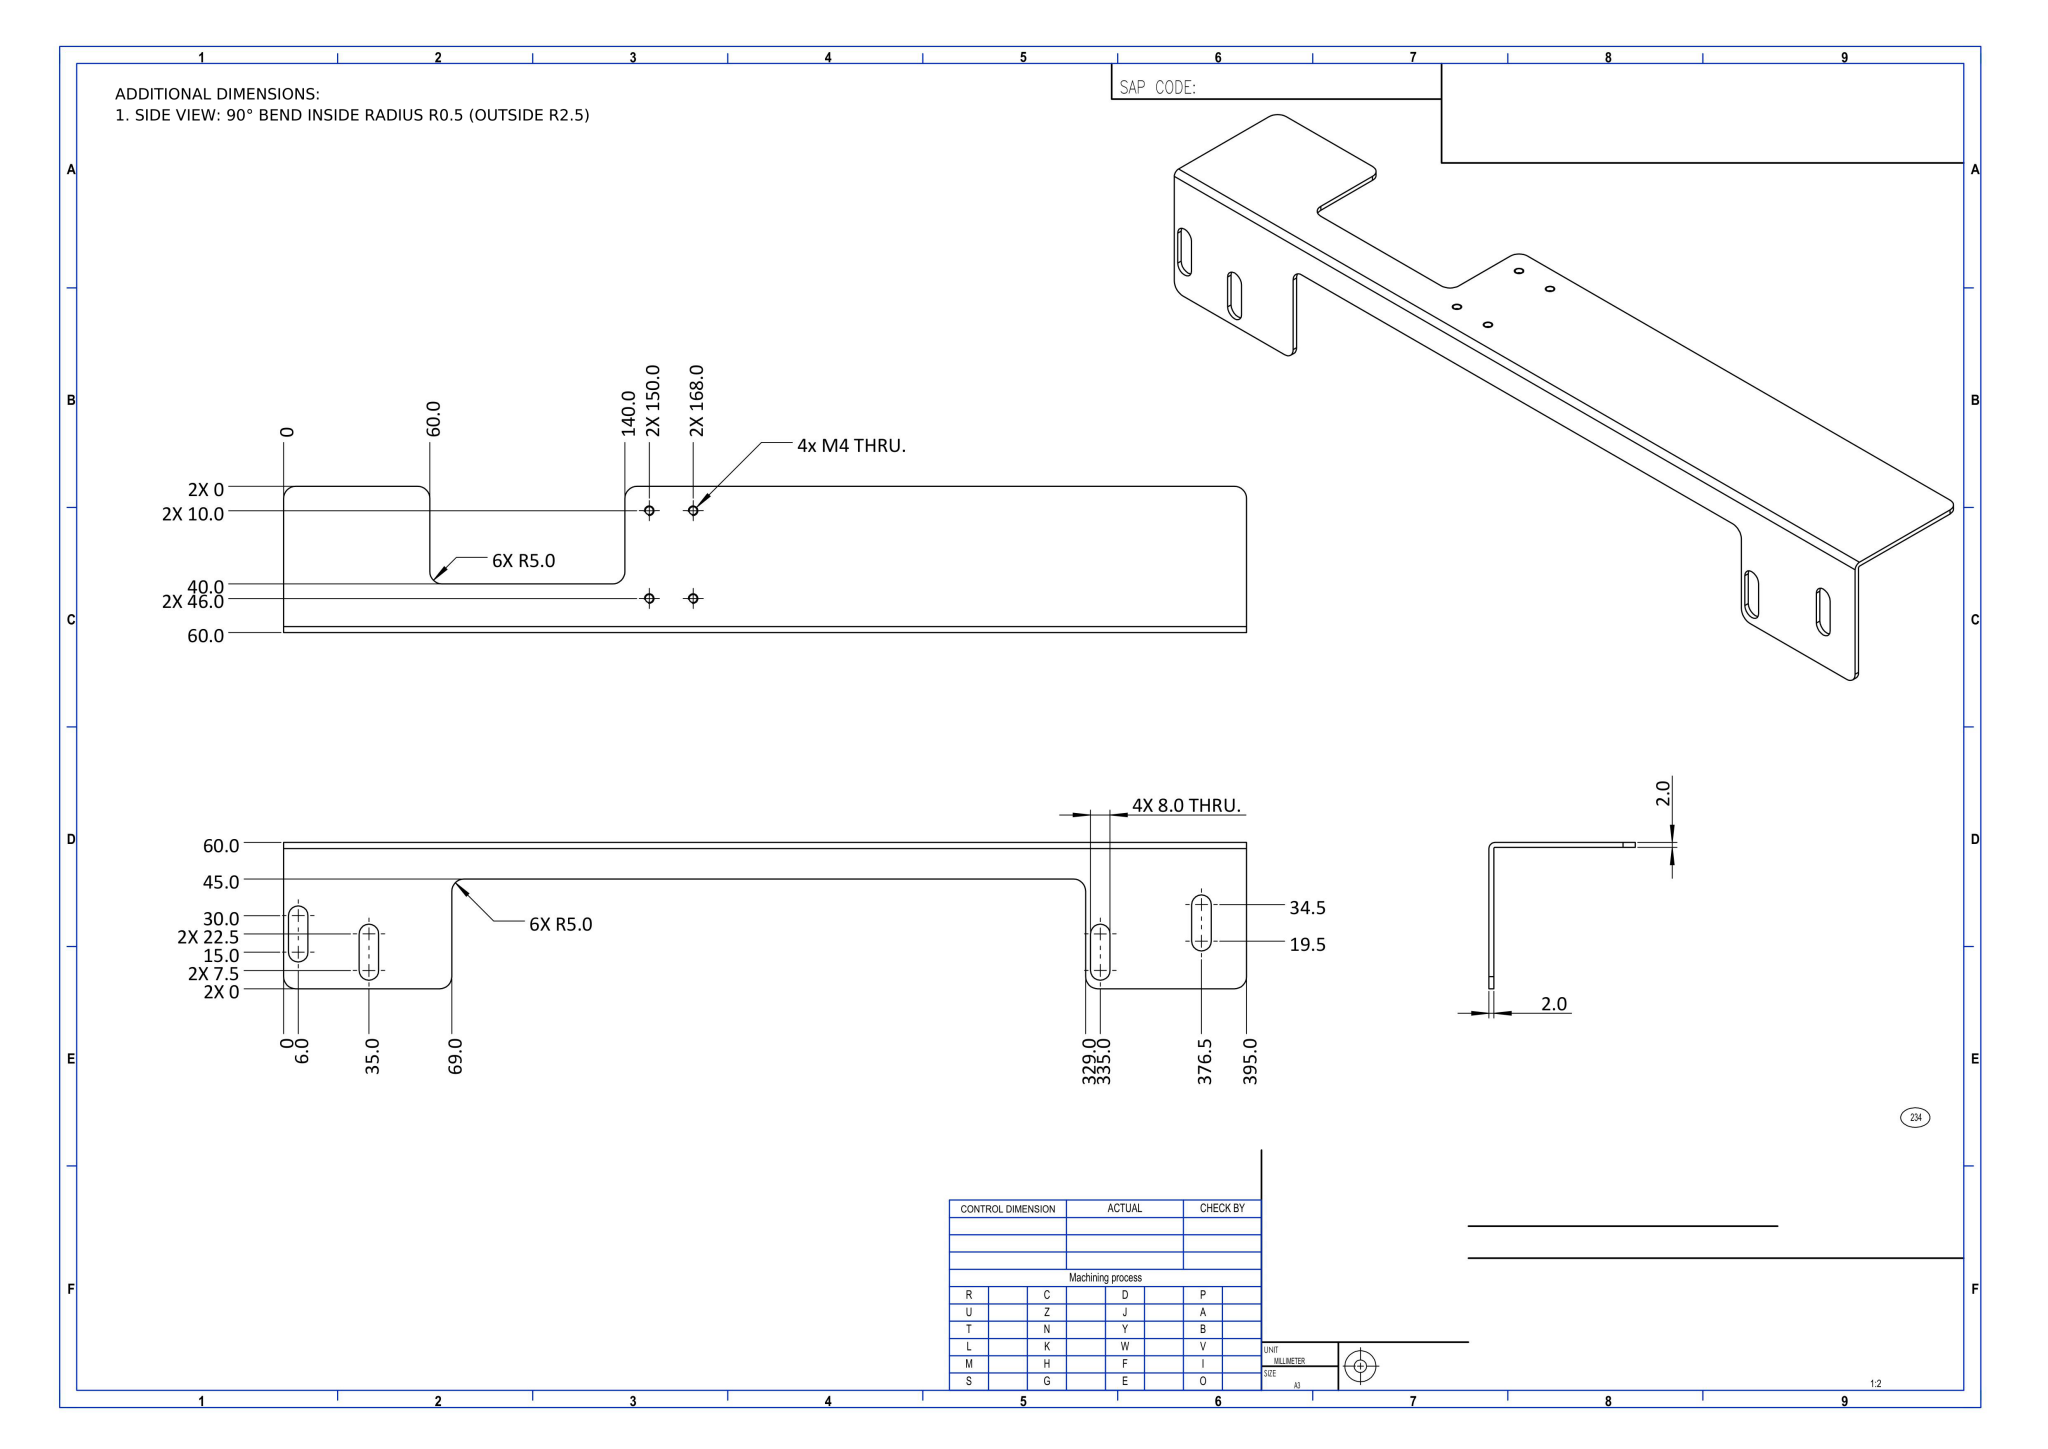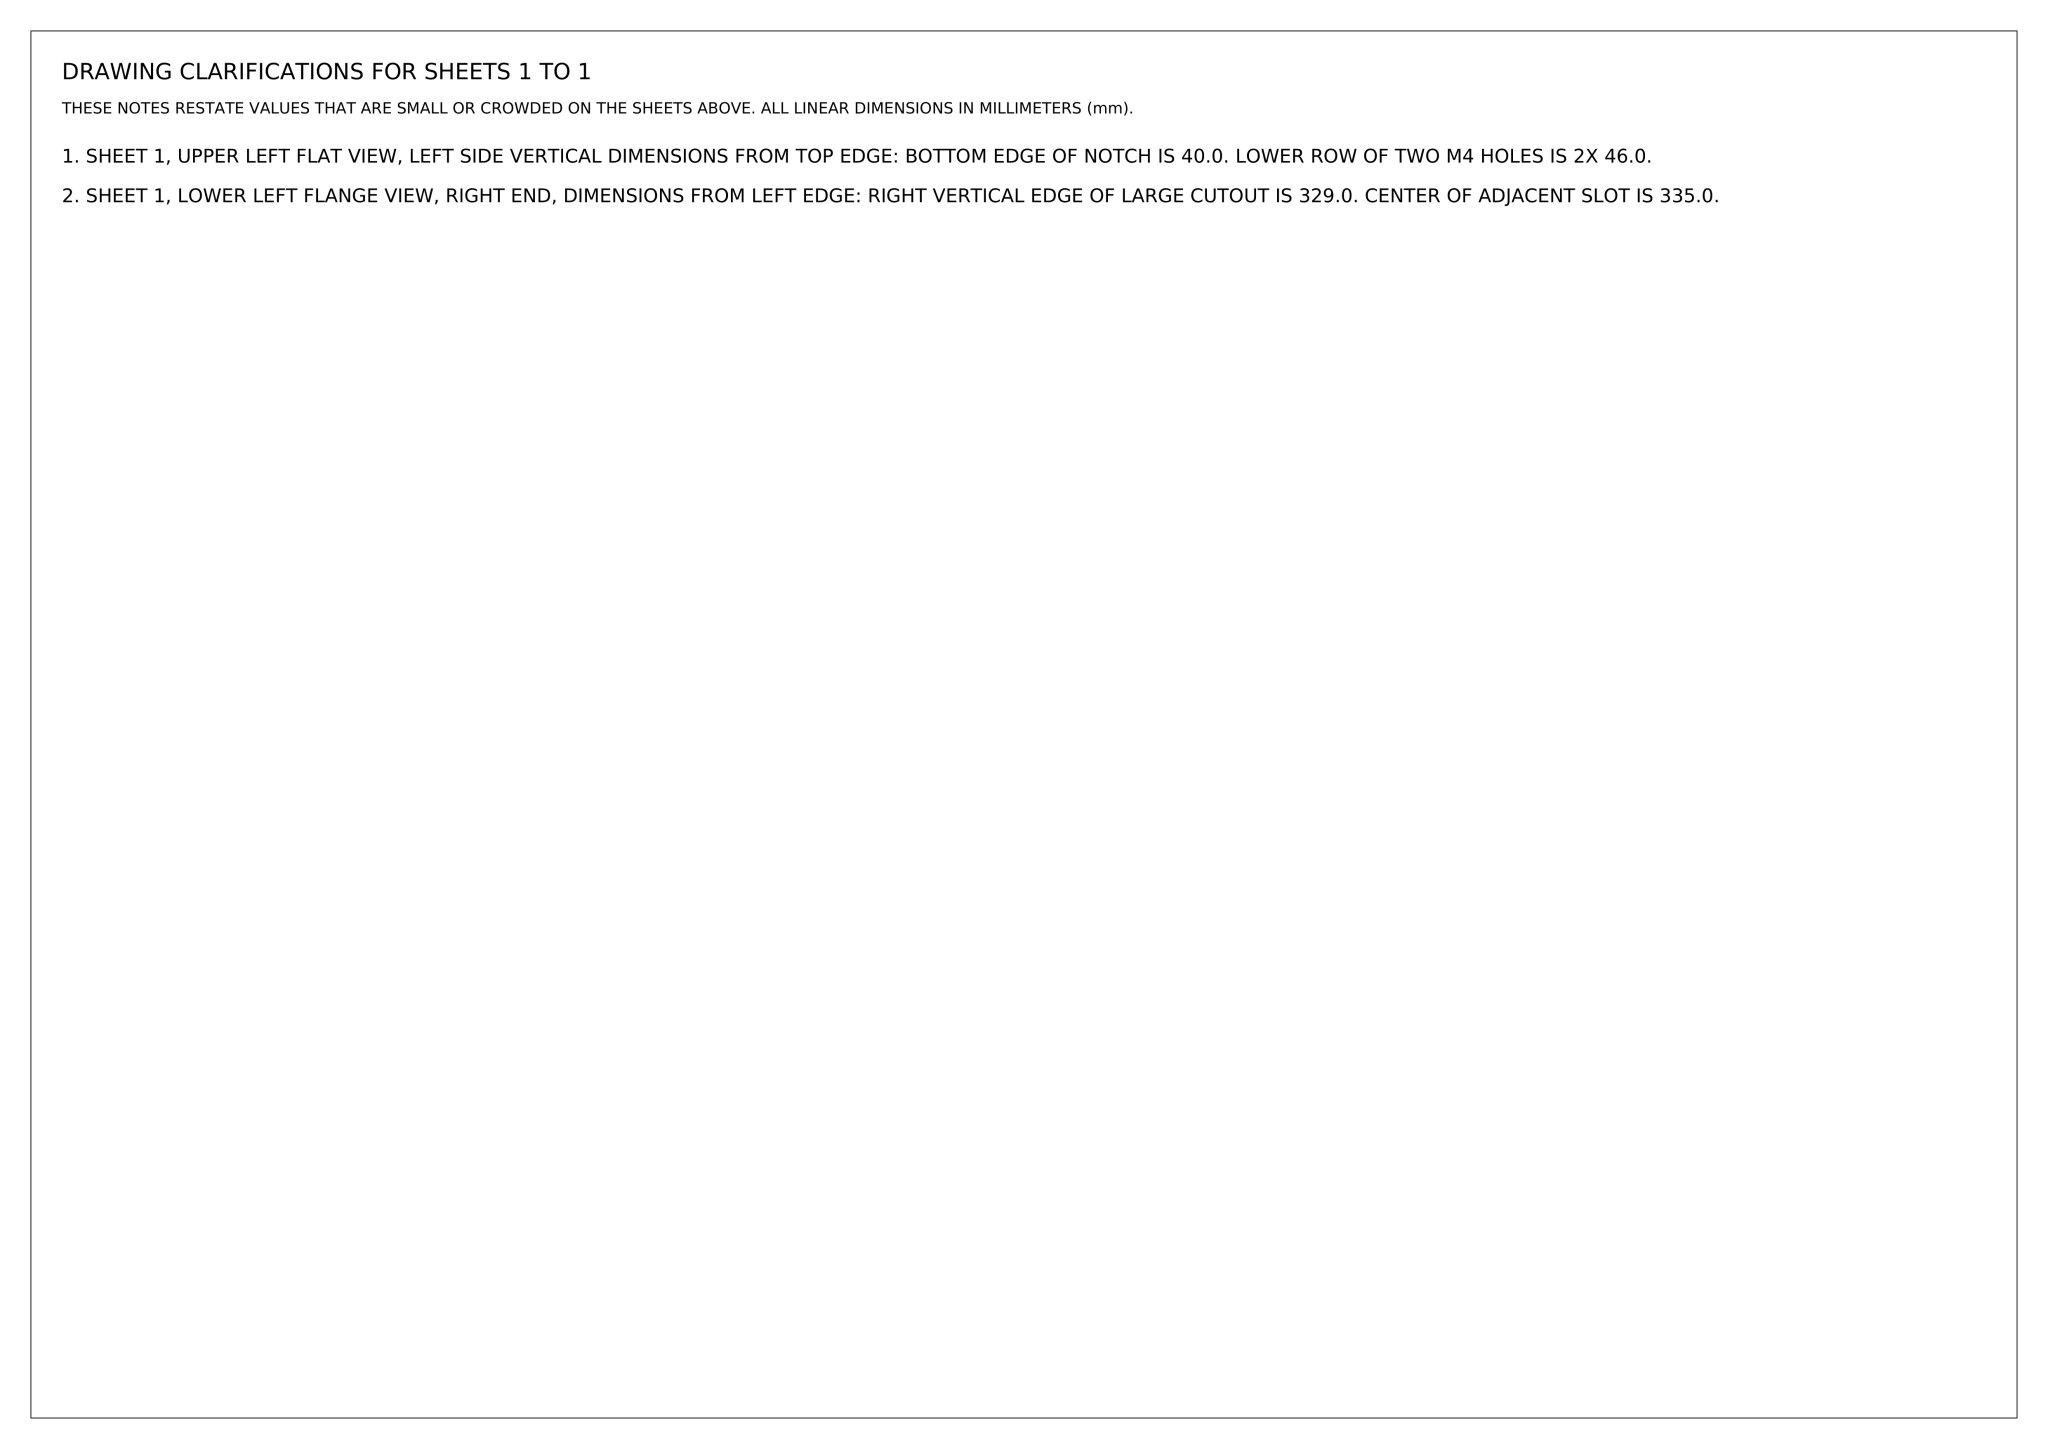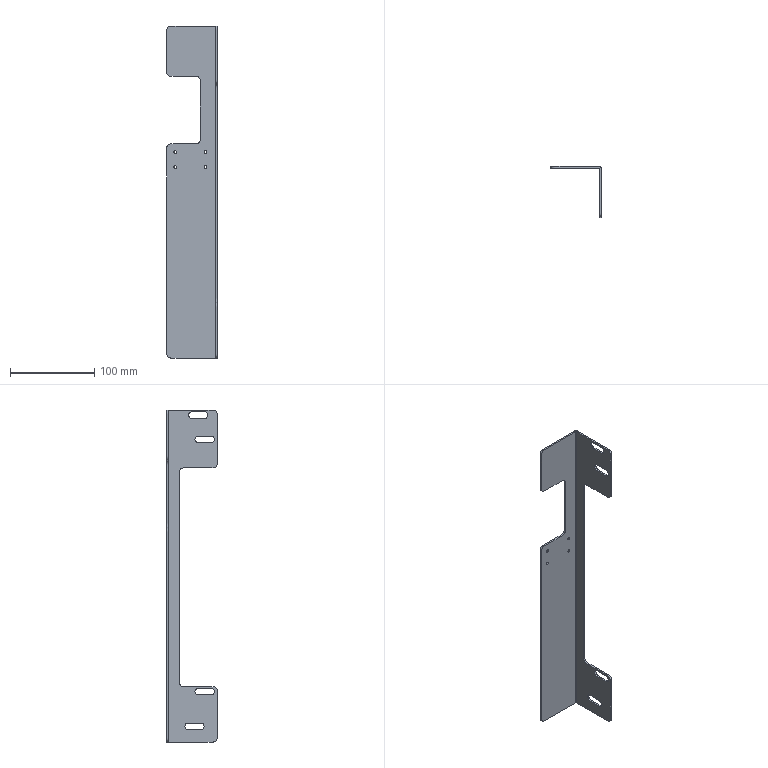Part | NX | mm | 1 solid | 54 faces | box 60 x 60 x 395 mm | volume 61438 mm3 | cylinder 30 | plane 24 | commonest cylinder face diameters 10 x12 3.3 x8 8 x8 5 x1 1 x1